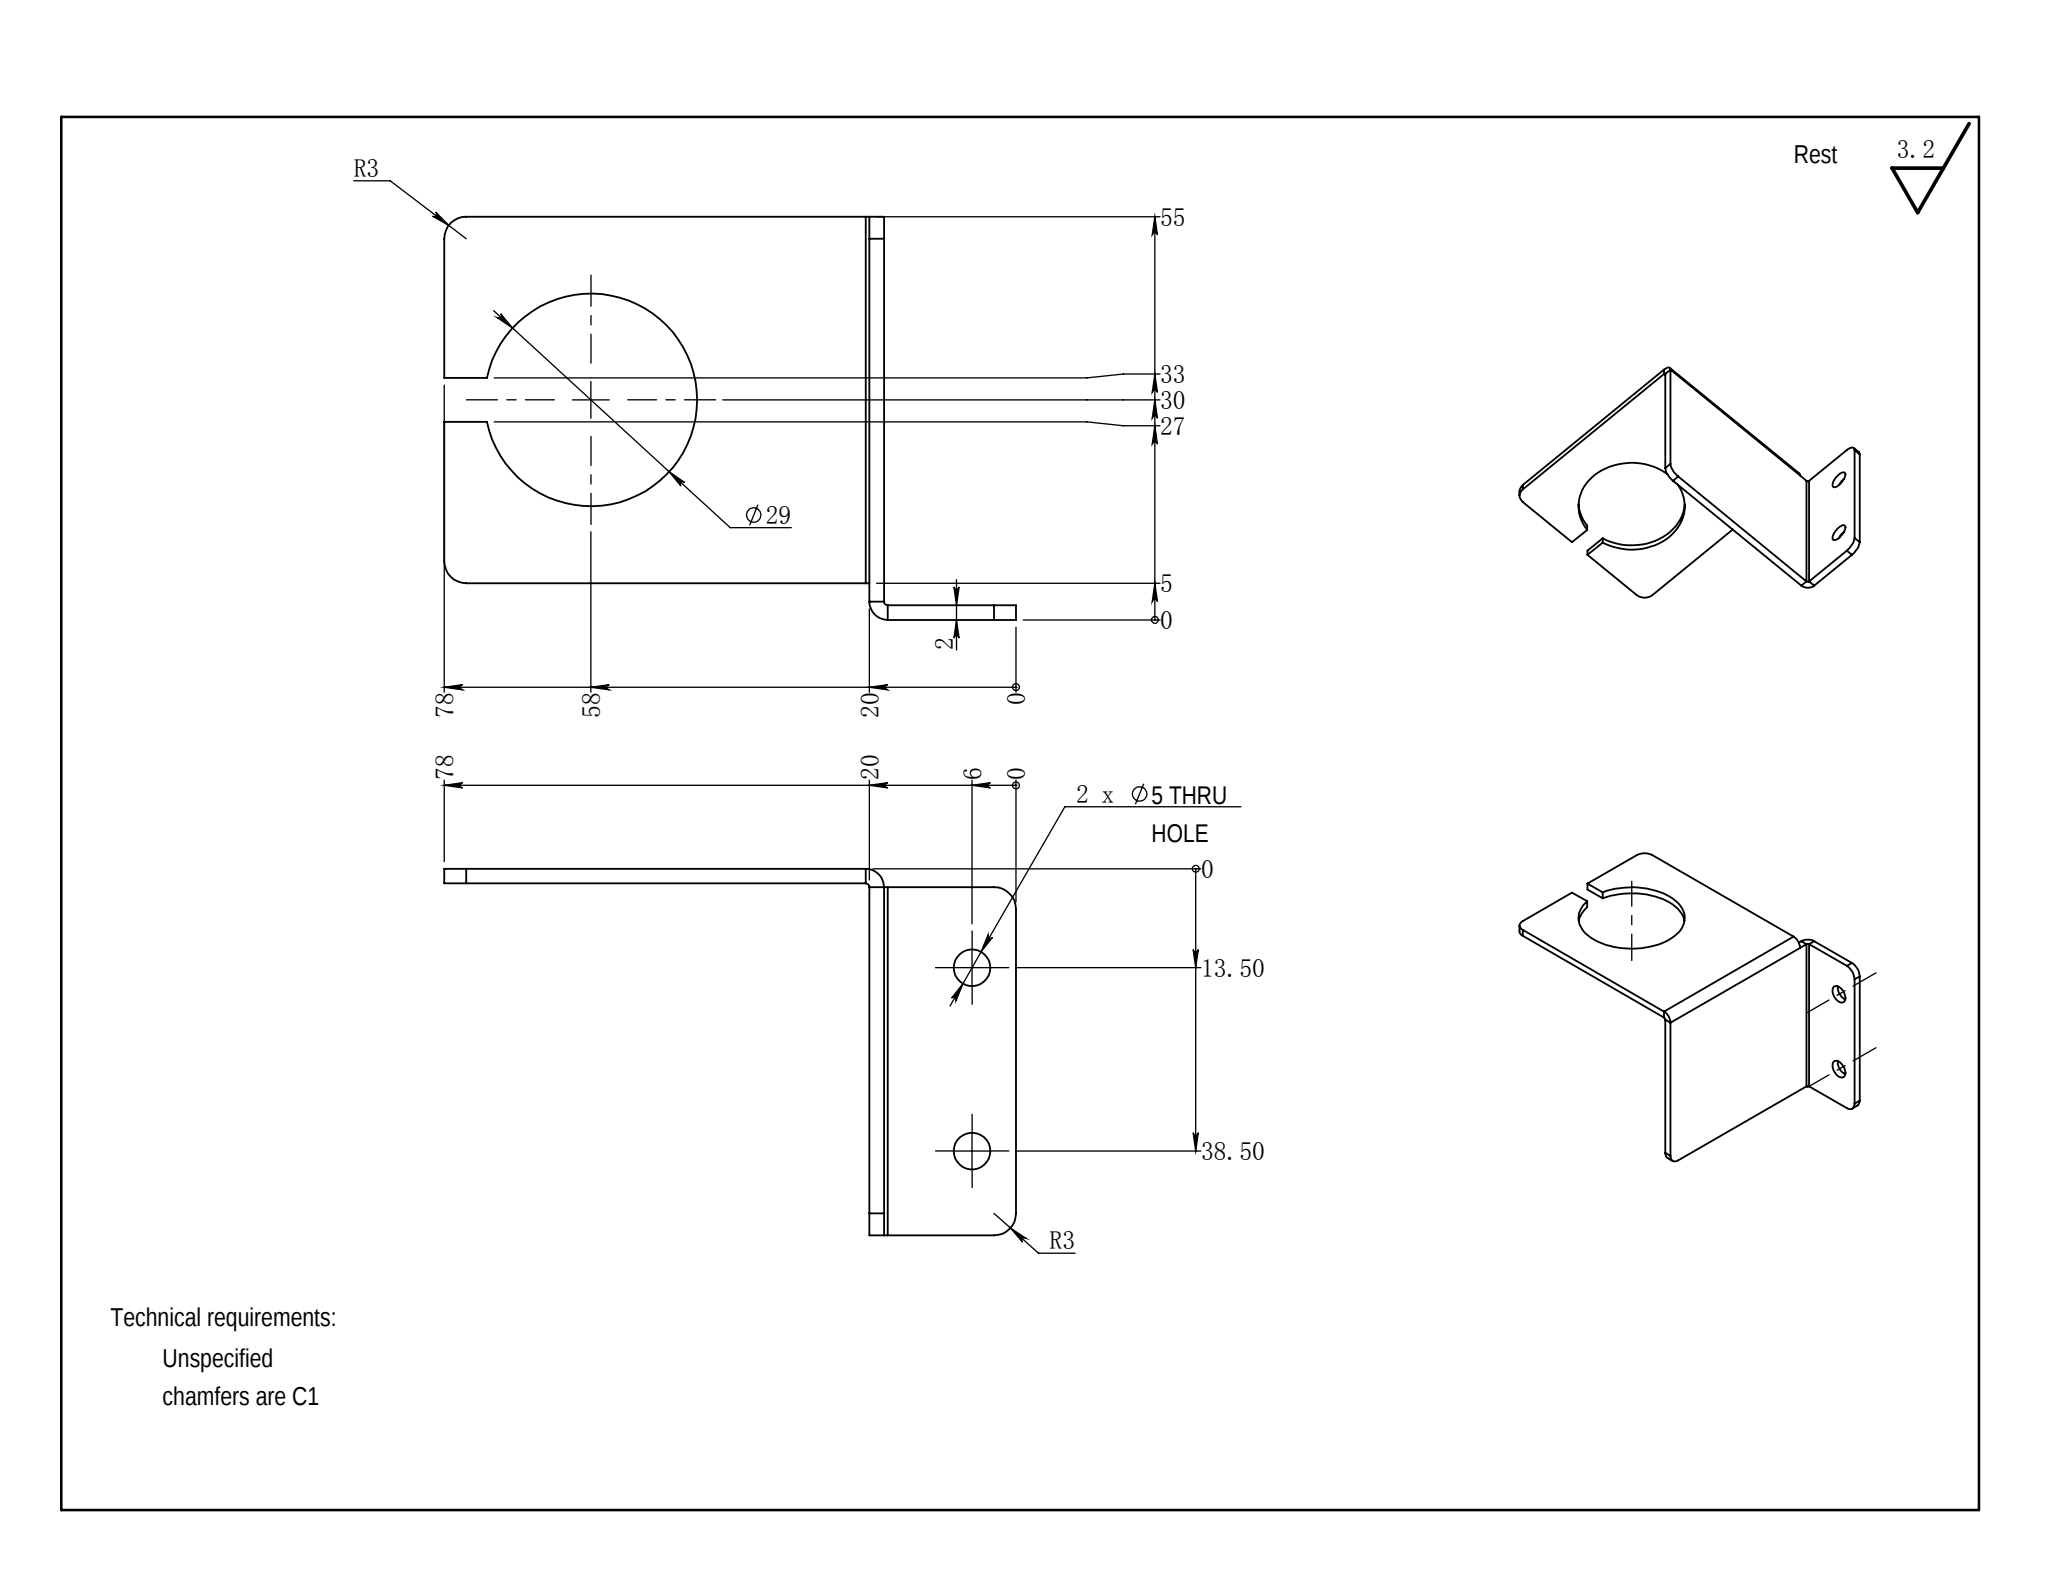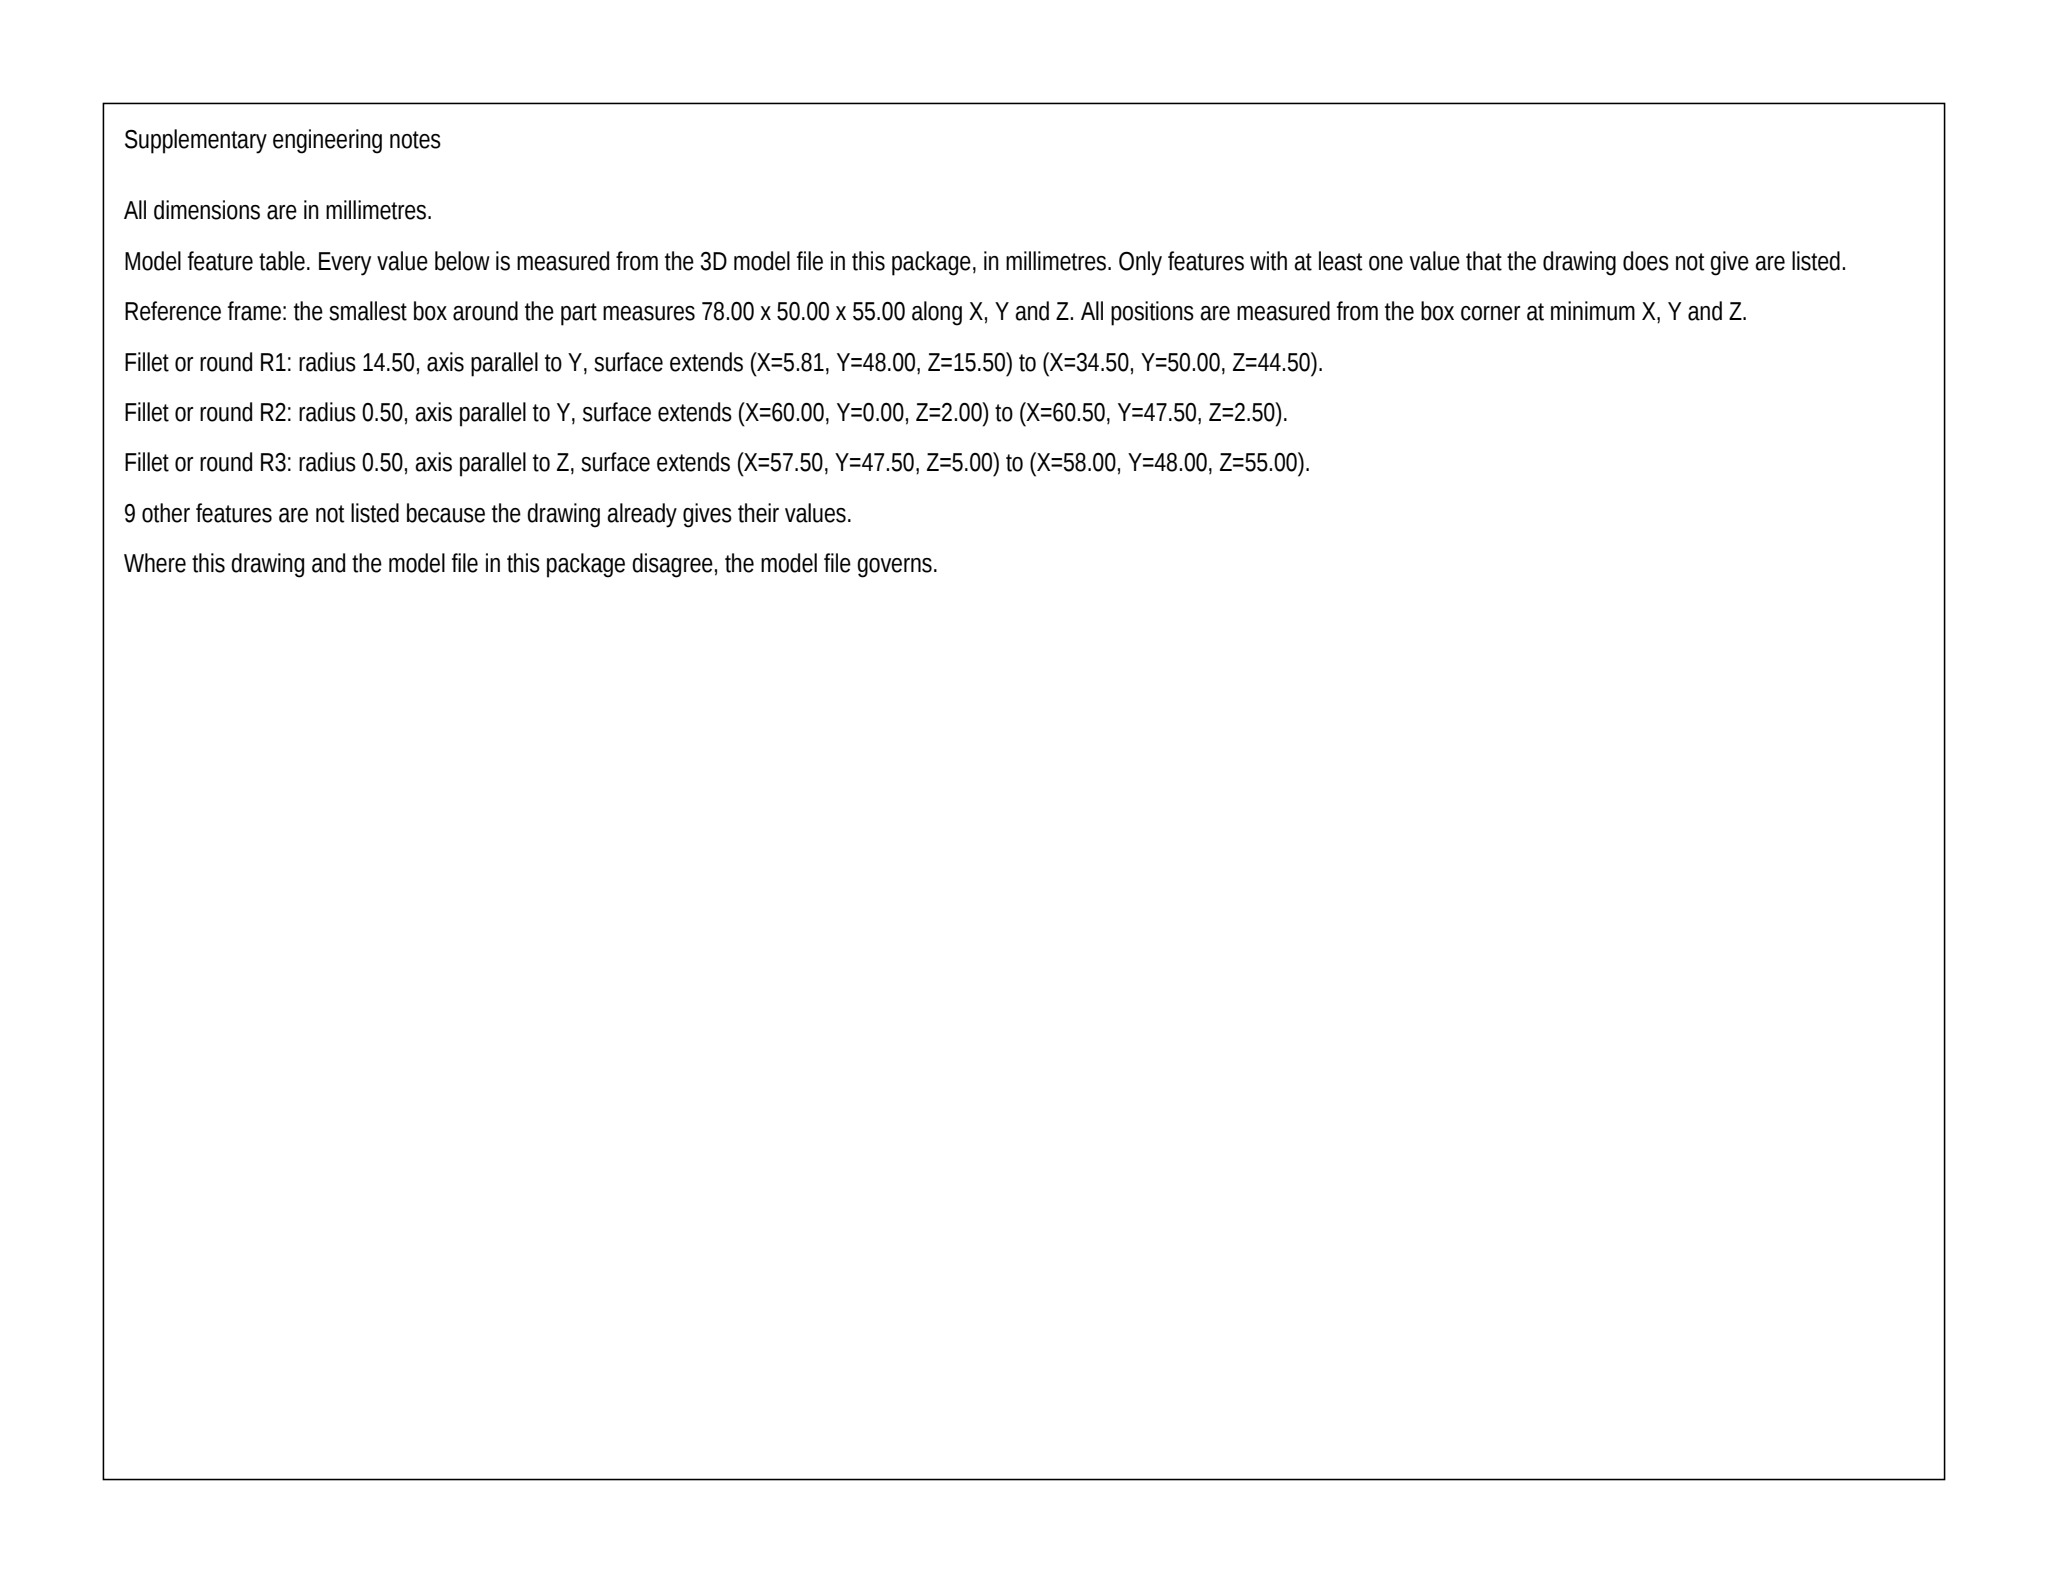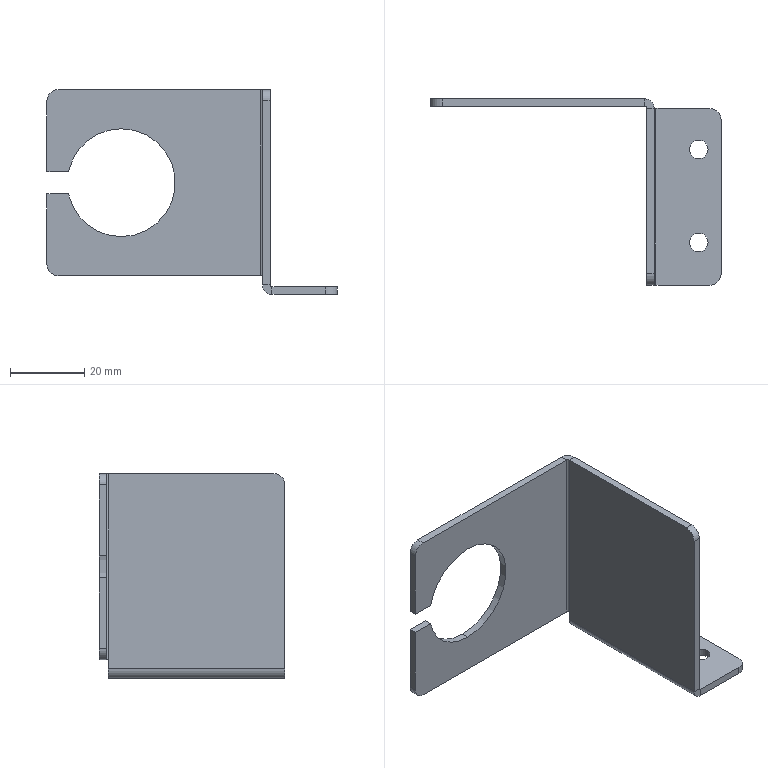Part | SolidWorks | mm | 1 solid | 38 faces | box 78 x 50 x 55 mm | volume 11373 mm3 | plane 22 | cylinder 16 | commonest cylinder face diameters 5 x6 6 x5 29 x3 1 x2
Drawing notes:
OVERALL WIDTH (Y) 50 FROM 0 DATUM AT TOP EDGE, LOWER VIEW | from the solid: bbox_xyz Y=50; Y planes at 0 and 50
UNSPECIFIED BEND RADII: R0.5 INSIDE, R2.5 OUTSIDE (2 THK) | from the solid: Y planes 47.5/50 give 2.5 outer offset on 2 thk wall
BENT WALL & BOTTOM FLANGE 47.5 WIDE (Y), SET BACK 2.5 FROM TOP FACE | from the solid: Y planes at 0 and 47.5 (3 faces each); 50-47.5=2.5